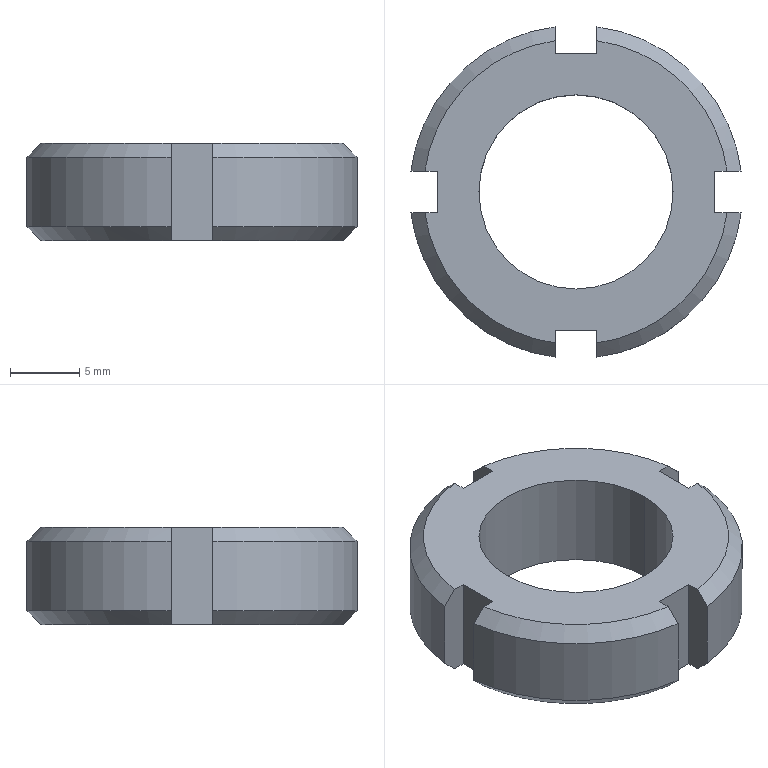Component | SolidWorks | 16RoundNutM14X1.5-1 | 1 solid | 28 faces | box 23.81 x 23.81 x 7 mm | volume 1863 mm3 | plane 14 | cone 8 | cylinder 6 | commonest cylinder face diameters 24 x4 14 x2
build123d program:
from build123d import *

# Parameters (mm, degrees)
SKETCH1_R              = 12
BOSS_EXTRUDE1_DEPTH    = 7
CHAMFER1_SIZE          = 1
M14X1_5_TAPPED_HOLE1_D = 14
SKETCH4_W              = 3
SKETCH4_H              = 4
CUT_EXTRUDE1_DEPTH     = 8
CIRPATTERN1_COUNT      = 4


with BuildPart() as part:
    # Sketch1 → Boss-Extrude1 (new body)
    with BuildSketch(Plane.XY):
        Circle(SKETCH1_R)
    extrude(amount=BOSS_EXTRUDE1_DEPTH)

    # Chamfer1
    chamfer1_edges = [part.edges().sort_by_distance(p)[0] for p in [
        (-12, 0, 0),
        (-12, 0, 7),
    ]]
    chamfer(chamfer1_edges, length=CHAMFER1_SIZE)

    # M14x1.5 Tapped Hole1 (through all)
    with Locations(Plane.XY.offset(7)):
        with Locations((0, 0)):
            Hole(M14X1_5_TAPPED_HOLE1_D / 2)

    # Sketch4 → Cut-Extrude1 (cut)
    with BuildSketch(Plane.XY):
        with Locations((0, 12)):
            Rectangle(SKETCH4_W, SKETCH4_H)
    cut_extrude1 = extrude(amount=CUT_EXTRUDE1_DEPTH, mode=Mode.SUBTRACT)

    # CirPattern1: Cut-Extrude1 ×4 about axis
    cirpattern1_axis = Axis((0, 0, 0), (0, 0, 1))
    for i in range(1, CIRPATTERN1_COUNT):
        add(cut_extrude1.rotate(cirpattern1_axis, i * 360 / CIRPATTERN1_COUNT), mode=Mode.SUBTRACT)


solid = part.part

# Placed as in the assembly
solid = solid.moved(Location((33.957, -55.224, 390), (0, 0, 0)))
STEP:
#1=COLOUR_RGB('',0.7922,0.8196,0.9333);
#2=FILL_AREA_STYLE_COLOUR('',#1);
#3=FILL_AREA_STYLE('',(#2));
#4=SURFACE_STYLE_FILL_AREA(#3);
#5=SURFACE_SIDE_STYLE('',(#4));
#6=SURFACE_STYLE_USAGE(.BOTH.,#5);
#7=PRESENTATION_STYLE_ASSIGNMENT((#6));
#8=CARTESIAN_POINT('',(1.061,-2.174,15.354));
#9=VERTEX_POINT('',#8);
#10=CARTESIAN_POINT('',(1.612,-2.174,15.354));
#11=VERTEX_POINT('',#10);
#12=CARTESIAN_POINT('',(1.337,-2.174,15.354));
#13=DIRECTION('',(0.,0.,1.));
#14=DIRECTION('',(1.,0.,0.));
#15=AXIS2_PLACEMENT_3D('',#12,#13,#14);
#16=CIRCLE('',#15,0.2756);
#17=EDGE_CURVE('',#9,#11,#16,.T.);
#18=ORIENTED_EDGE('',*,*,#17,.F.);
#19=CARTESIAN_POINT('',(1.061,-2.174,15.63));
#20=VERTEX_POINT('',#19);
#21=CARTESIAN_POINT('',(1.061,-2.174,15.63));
#22=DIRECTION('',(0.,0.,1.));
#23=VECTOR('',#22,39.37);
#24=LINE('',#21,#23);
#25=EDGE_CURVE('',#9,#20,#24,.T.);
#26=ORIENTED_EDGE('',*,*,#25,.T.);
#27=CARTESIAN_POINT('',(1.612,-2.174,15.63));
#28=VERTEX_POINT('',#27);
#29=CARTESIAN_POINT('',(1.337,-2.174,15.63));
#30=DIRECTION('',(0.,0.,1.));
#31=DIRECTION('',(1.,0.,0.));
#32=AXIS2_PLACEMENT_3D('',#29,#30,#31);
#33=CIRCLE('',#32,0.2756);
#34=EDGE_CURVE('',#20,#28,#33,.T.);
#35=ORIENTED_EDGE('',*,*,#34,.T.);
#36=CARTESIAN_POINT('',(1.612,-2.174,15.63));
#37=DIRECTION('',(0.,0.,1.));
#38=VECTOR('',#37,39.37);
#39=LINE('',#36,#38);
#40=EDGE_CURVE('',#11,#28,#39,.T.);
#41=ORIENTED_EDGE('',*,*,#40,.F.);
#42=EDGE_LOOP('',(#18,#26,#35,#41));
#43=FACE_OUTER_BOUND('',#42,.T.);
#44=CARTESIAN_POINT('',(1.337,-2.174,15.63));
#45=DIRECTION('',(0.,0.,1.));
#46=DIRECTION('',(1.,0.,0.));
#47=AXIS2_PLACEMENT_3D('',#44,#45,#46);
#48=CYLINDRICAL_SURFACE('',#47,0.2756);
#49=ADVANCED_FACE('',(#43),#48,.F.);
#50=CARTESIAN_POINT('',(1.278,-2.643,15.591));
#51=VERTEX_POINT('',#50);
#52=CARTESIAN_POINT('',(1.278,-2.643,15.394));
#53=VERTEX_POINT('',#52);
#54=CARTESIAN_POINT('',(1.278,-2.643,15.63));
#55=DIRECTION('',(0.,0.,-1.));
#56=VECTOR('',#55,39.37);
#57=LINE('',#54,#56);
#58=EDGE_CURVE('',#51,#53,#57,.T.);
#59=ORIENTED_EDGE('',*,*,#58,.F.);
#60=CARTESIAN_POINT('',(0.8682,-2.233,15.591));
#61=VERTEX_POINT('',#60);
#62=CARTESIAN_POINT('',(1.337,-2.174,15.591));
#63=DIRECTION('',(0.,0.,-1.));
#64=DIRECTION('',(1.,0.,0.));
#65=AXIS2_PLACEMENT_3D('',#62,#63,#64);
#66=CIRCLE('',#65,0.4724);
#67=EDGE_CURVE('',#51,#61,#66,.T.);
#68=ORIENTED_EDGE('',*,*,#67,.T.);
#69=CARTESIAN_POINT('',(0.8682,-2.233,15.394));
#70=VERTEX_POINT('',#69);
#71=CARTESIAN_POINT('',(0.8682,-2.233,15.63));
#72=DIRECTION('',(0.,0.,1.));
#73=VECTOR('',#72,39.37);
#74=LINE('',#71,#73);
#75=EDGE_CURVE('',#70,#61,#74,.T.);
#76=ORIENTED_EDGE('',*,*,#75,.F.);
#77=CARTESIAN_POINT('',(1.337,-2.174,15.394));
#78=DIRECTION('',(0.,0.,1.));
#79=DIRECTION('',(1.,0.,0.));
#80=AXIS2_PLACEMENT_3D('',#77,#78,#79);
#81=CIRCLE('',#80,0.4724);
#82=EDGE_CURVE('',#70,#53,#81,.T.);
#83=ORIENTED_EDGE('',*,*,#82,.T.);
#84=EDGE_LOOP('',(#59,#68,#76,#83));
#85=FACE_OUTER_BOUND('',#84,.T.);
#86=CARTESIAN_POINT('',(1.337,-2.174,15.63));
#87=DIRECTION('',(0.,0.,-1.));
#88=DIRECTION('',(-1.,0.,0.));
#89=AXIS2_PLACEMENT_3D('',#86,#87,#88);
#90=CYLINDRICAL_SURFACE('',#89,0.4724);
#91=ADVANCED_FACE('',(#85),#90,.T.);
#92=CARTESIAN_POINT('',(1.396,-2.643,15.394));
#93=VERTEX_POINT('',#92);
#94=CARTESIAN_POINT('',(1.396,-2.643,15.591));
#95=VERTEX_POINT('',#94);
#96=CARTESIAN_POINT('',(1.396,-2.643,15.63));
#97=DIRECTION('',(0.,0.,1.));
#98=VECTOR('',#97,39.37);
#99=LINE('',#96,#98);
#100=EDGE_CURVE('',#93,#95,#99,.T.);
#101=ORIENTED_EDGE('',*,*,#100,.F.);
#102=CARTESIAN_POINT('',(1.806,-2.233,15.394));
#103=VERTEX_POINT('',#102);
#104=CARTESIAN_POINT('',(1.337,-2.174,15.394));
#105=DIRECTION('',(0.,0.,1.));
#106=DIRECTION('',(1.,0.,0.));
#107=AXIS2_PLACEMENT_3D('',#104,#105,#106);
#108=CIRCLE('',#107,0.4724);
#109=EDGE_CURVE('',#93,#103,#108,.T.);
#110=ORIENTED_EDGE('',*,*,#109,.T.);
#111=CARTESIAN_POINT('',(1.806,-2.233,15.591));
#112=VERTEX_POINT('',#111);
#113=CARTESIAN_POINT('',(1.806,-2.233,15.63));
#114=DIRECTION('',(0.,0.,-1.));
#115=VECTOR('',#114,39.37);
#116=LINE('',#113,#115);
#117=EDGE_CURVE('',#112,#103,#116,.T.);
#118=ORIENTED_EDGE('',*,*,#117,.F.);
#119=CARTESIAN_POINT('',(1.337,-2.174,15.591));
#120=DIRECTION('',(0.,0.,-1.));
#121=DIRECTION('',(1.,0.,0.));
#122=AXIS2_PLACEMENT_3D('',#119,#120,#121);
#123=CIRCLE('',#122,0.4724);
#124=EDGE_CURVE('',#112,#95,#123,.T.);
#125=ORIENTED_EDGE('',*,*,#124,.T.);
#126=EDGE_LOOP('',(#101,#110,#118,#125));
#127=FACE_OUTER_BOUND('',#126,.T.);
#128=CARTESIAN_POINT('',(1.337,-2.174,15.63));
#129=DIRECTION('',(0.,0.,-1.));
#130=DIRECTION('',(-1.,0.,0.));
#131=AXIS2_PLACEMENT_3D('',#128,#129,#130);
#132=CYLINDRICAL_SURFACE('',#131,0.4724);
#133=ADVANCED_FACE('',(#127),#132,.T.);
#134=CARTESIAN_POINT('',(0.8682,-2.115,15.591));
#135=VERTEX_POINT('',#134);
#136=CARTESIAN_POINT('',(0.8682,-2.115,15.394));
#137=VERTEX_POINT('',#136);
#138=CARTESIAN_POINT('',(0.8682,-2.115,15.63));
#139=DIRECTION('',(0.,0.,-1.));
#140=VECTOR('',#139,39.37);
#141=LINE('',#138,#140);
#142=EDGE_CURVE('',#135,#137,#141,.T.);
#143=ORIENTED_EDGE('',*,*,#142,.F.);
#144=CARTESIAN_POINT('',(1.278,-1.705,15.591));
#145=VERTEX_POINT('',#144);
#146=CARTESIAN_POINT('',(1.337,-2.174,15.591));
#147=DIRECTION('',(0.,0.,-1.));
#148=DIRECTION('',(1.,0.,0.));
#149=AXIS2_PLACEMENT_3D('',#146,#147,#148);
#150=CIRCLE('',#149,0.4724);
#151=EDGE_CURVE('',#135,#145,#150,.T.);
#152=ORIENTED_EDGE('',*,*,#151,.T.);
#153=CARTESIAN_POINT('',(1.278,-1.705,15.394));
#154=VERTEX_POINT('',#153);
#155=CARTESIAN_POINT('',(1.278,-1.705,15.63));
#156=DIRECTION('',(0.,0.,1.));
#157=VECTOR('',#156,39.37);
#158=LINE('',#155,#157);
#159=EDGE_CURVE('',#154,#145,#158,.T.);
#160=ORIENTED_EDGE('',*,*,#159,.F.);
#161=CARTESIAN_POINT('',(1.337,-2.174,15.394));
#162=DIRECTION('',(0.,0.,1.));
#163=DIRECTION('',(1.,0.,0.));
#164=AXIS2_PLACEMENT_3D('',#161,#162,#163);
#165=CIRCLE('',#164,0.4724);
#166=EDGE_CURVE('',#154,#137,#165,.T.);
#167=ORIENTED_EDGE('',*,*,#166,.T.);
#168=EDGE_LOOP('',(#143,#152,#160,#167));
#169=FACE_OUTER_BOUND('',#168,.T.);
#170=CARTESIAN_POINT('',(1.337,-2.174,15.63));
#171=DIRECTION('',(0.,0.,-1.));
#172=DIRECTION('',(-1.,0.,0.));
#173=AXIS2_PLACEMENT_3D('',#170,#171,#172);
#174=CYLINDRICAL_SURFACE('',#173,0.4724);
#175=ADVANCED_FACE('',(#169),#174,.T.);
#176=CARTESIAN_POINT('',(1.337,-2.174,15.63));
#177=DIRECTION('',(0.,0.,1.));
#178=DIRECTION('',(1.,0.,0.));
#179=AXIS2_PLACEMENT_3D('',#176,#177,#178);
#180=CIRCLE('',#179,0.2756);
#181=EDGE_CURVE('',#28,#20,#180,.T.);
#182=ORIENTED_EDGE('',*,*,#181,.F.);
#183=ORIENTED_EDGE('',*,*,#34,.F.);
#184=EDGE_LOOP('',(#182,#183));
#185=FACE_BOUND('',#184,.T.);
#186=CARTESIAN_POINT('',(0.9079,-2.233,15.63));
#187=VERTEX_POINT('',#186);
#188=CARTESIAN_POINT('',(1.278,-2.603,15.63));
#189=VERTEX_POINT('',#188);
#190=CARTESIAN_POINT('',(1.337,-2.174,15.63));
#191=DIRECTION('',(0.,0.,1.));
#192=DIRECTION('',(1.,0.,0.));
#193=AXIS2_PLACEMENT_3D('',#190,#191,#192);
#194=CIRCLE('',#193,0.4331);
#195=EDGE_CURVE('',#187,#189,#194,.T.);
#196=ORIENTED_EDGE('',*,*,#195,.T.);
#197=CARTESIAN_POINT('',(1.278,-2.568,15.63));
#198=VERTEX_POINT('',#197);
#199=CARTESIAN_POINT('',(1.278,-2.174,15.63));
#200=DIRECTION('',(0.,1.,0.));
#201=VECTOR('',#200,39.37);
#202=LINE('',#199,#201);
#203=EDGE_CURVE('',#189,#198,#202,.T.);
#204=ORIENTED_EDGE('',*,*,#203,.T.);
#205=CARTESIAN_POINT('',(1.396,-2.568,15.63));
#206=VERTEX_POINT('',#205);
#207=CARTESIAN_POINT('',(1.337,-2.568,15.63));
#208=DIRECTION('',(1.,0.,0.));
#209=VECTOR('',#208,39.37);
#210=LINE('',#207,#209);
#211=EDGE_CURVE('',#198,#206,#210,.T.);
#212=ORIENTED_EDGE('',*,*,#211,.T.);
#213=CARTESIAN_POINT('',(1.396,-2.603,15.63));
#214=VERTEX_POINT('',#213);
#215=CARTESIAN_POINT('',(1.396,-2.174,15.63));
#216=DIRECTION('',(-0.,-1.,0.));
#217=VECTOR('',#216,39.37);
#218=LINE('',#215,#217);
#219=EDGE_CURVE('',#206,#214,#218,.T.);
#220=ORIENTED_EDGE('',*,*,#219,.T.);
#221=CARTESIAN_POINT('',(1.766,-2.233,15.63));
#222=VERTEX_POINT('',#221);
#223=CARTESIAN_POINT('',(1.337,-2.174,15.63));
#224=DIRECTION('',(0.,0.,1.));
#225=DIRECTION('',(1.,0.,0.));
#226=AXIS2_PLACEMENT_3D('',#223,#224,#225);
#227=CIRCLE('',#226,0.4331);
#228=EDGE_CURVE('',#214,#222,#227,.T.);
#229=ORIENTED_EDGE('',*,*,#228,.T.);
#230=CARTESIAN_POINT('',(1.731,-2.233,15.63));
#231=VERTEX_POINT('',#230);
#232=CARTESIAN_POINT('',(1.337,-2.233,15.63));
#233=DIRECTION('',(-1.,0.,0.));
#234=VECTOR('',#233,39.37);
#235=LINE('',#232,#234);
#236=EDGE_CURVE('',#222,#231,#235,.T.);
#237=ORIENTED_EDGE('',*,*,#236,.T.);
#238=CARTESIAN_POINT('',(1.731,-2.115,15.63));
#239=VERTEX_POINT('',#238);
#240=CARTESIAN_POINT('',(1.731,-2.174,15.63));
#241=DIRECTION('',(0.,1.,0.));
#242=VECTOR('',#241,39.37);
#243=LINE('',#240,#242);
#244=EDGE_CURVE('',#231,#239,#243,.T.);
#245=ORIENTED_EDGE('',*,*,#244,.T.);
#246=CARTESIAN_POINT('',(1.766,-2.115,15.63));
#247=VERTEX_POINT('',#246);
#248=CARTESIAN_POINT('',(1.337,-2.115,15.63));
#249=DIRECTION('',(1.,-0.,0.));
#250=VECTOR('',#249,39.37);
#251=LINE('',#248,#250);
#252=EDGE_CURVE('',#239,#247,#251,.T.);
#253=ORIENTED_EDGE('',*,*,#252,.T.);
#254=CARTESIAN_POINT('',(1.396,-1.745,15.63));
#255=VERTEX_POINT('',#254);
#256=CARTESIAN_POINT('',(1.337,-2.174,15.63));
#257=DIRECTION('',(0.,0.,1.));
#258=DIRECTION('',(1.,0.,0.));
#259=AXIS2_PLACEMENT_3D('',#256,#257,#258);
#260=CIRCLE('',#259,0.4331);
#261=EDGE_CURVE('',#247,#255,#260,.T.);
#262=ORIENTED_EDGE('',*,*,#261,.T.);
#263=CARTESIAN_POINT('',(1.396,-1.78,15.63));
#264=VERTEX_POINT('',#263);
#265=CARTESIAN_POINT('',(1.396,-2.174,15.63));
#266=DIRECTION('',(-0.,-1.,0.));
#267=VECTOR('',#266,39.37);
#268=LINE('',#265,#267);
#269=EDGE_CURVE('',#255,#264,#268,.T.);
#270=ORIENTED_EDGE('',*,*,#269,.T.);
#271=CARTESIAN_POINT('',(1.278,-1.78,15.63));
#272=VERTEX_POINT('',#271);
#273=CARTESIAN_POINT('',(1.337,-1.78,15.63));
#274=DIRECTION('',(-1.,0.,0.));
#275=VECTOR('',#274,39.37);
#276=LINE('',#273,#275);
#277=EDGE_CURVE('',#264,#272,#276,.T.);
#278=ORIENTED_EDGE('',*,*,#277,.T.);
#279=CARTESIAN_POINT('',(1.278,-1.745,15.63));
#280=VERTEX_POINT('',#279);
#281=CARTESIAN_POINT('',(1.278,-2.174,15.63));
#282=DIRECTION('',(0.,1.,0.));
#283=VECTOR('',#282,39.37);
#284=LINE('',#281,#283);
#285=EDGE_CURVE('',#272,#280,#284,.T.);
#286=ORIENTED_EDGE('',*,*,#285,.T.);
#287=CARTESIAN_POINT('',(0.9079,-2.115,15.63));
#288=VERTEX_POINT('',#287);
#289=CARTESIAN_POINT('',(1.337,-2.174,15.63));
#290=DIRECTION('',(0.,0.,1.));
#291=DIRECTION('',(1.,0.,0.));
#292=AXIS2_PLACEMENT_3D('',#289,#290,#291);
#293=CIRCLE('',#292,0.4331);
#294=EDGE_CURVE('',#280,#288,#293,.T.);
#295=ORIENTED_EDGE('',*,*,#294,.T.);
#296=CARTESIAN_POINT('',(0.9432,-2.115,15.63));
#297=VERTEX_POINT('',#296);
#298=CARTESIAN_POINT('',(1.337,-2.115,15.63));
#299=DIRECTION('',(1.,-0.,0.));
#300=VECTOR('',#299,39.37);
#301=LINE('',#298,#300);
#302=EDGE_CURVE('',#288,#297,#301,.T.);
#303=ORIENTED_EDGE('',*,*,#302,.T.);
#304=CARTESIAN_POINT('',(0.9432,-2.233,15.63));
#305=VERTEX_POINT('',#304);
#306=CARTESIAN_POINT('',(0.9432,-2.174,15.63));
#307=DIRECTION('',(-0.,-1.,0.));
#308=VECTOR('',#307,39.37);
#309=LINE('',#306,#308);
#310=EDGE_CURVE('',#297,#305,#309,.T.);
#311=ORIENTED_EDGE('',*,*,#310,.T.);
#312=CARTESIAN_POINT('',(1.337,-2.233,15.63));
#313=DIRECTION('',(-1.,0.,0.));
#314=VECTOR('',#313,39.37);
#315=LINE('',#312,#314);
#316=EDGE_CURVE('',#305,#187,#315,.T.);
#317=ORIENTED_EDGE('',*,*,#316,.T.);
#318=EDGE_LOOP('',(#196,#204,#212,#220,#229,#237,#245,#253,#262,#270,#278,#286,#295,#303,#311,#317));
#319=FACE_OUTER_BOUND('',#318,.T.);
#320=CARTESIAN_POINT('',(1.337,-2.174,15.63));
#321=DIRECTION('',(0.,0.,1.));
#322=DIRECTION('',(1.,0.,0.));
#323=AXIS2_PLACEMENT_3D('',#320,#321,#322);
#324=PLANE('',#323);
#325=ADVANCED_FACE('',(#185,#319),#324,.T.);
#326=CARTESIAN_POINT('',(1.337,-2.174,15.354));
#327=DIRECTION('',(0.,0.,1.));
#328=DIRECTION('',(1.,0.,0.));
#329=AXIS2_PLACEMENT_3D('',#326,#327,#328);
#330=CIRCLE('',#329,0.2756);
#331=EDGE_CURVE('',#11,#9,#330,.T.);
#332=ORIENTED_EDGE('',*,*,#331,.T.);
#333=ORIENTED_EDGE('',*,*,#17,.T.);
#334=EDGE_LOOP('',(#332,#333));
#335=FACE_BOUND('',#334,.T.);
#336=CARTESIAN_POINT('',(1.278,-2.568,15.354));
#337=VERTEX_POINT('',#336);
#338=CARTESIAN_POINT('',(1.278,-2.603,15.354));
#339=VERTEX_POINT('',#338);
#340=CARTESIAN_POINT('',(1.278,-2.568,15.354));
#341=DIRECTION('',(-0.,-1.,0.));
#342=VECTOR('',#341,39.37);
#343=LINE('',#340,#342);
#344=EDGE_CURVE('',#337,#339,#343,.T.);
#345=ORIENTED_EDGE('',*,*,#344,.T.);
#346=CARTESIAN_POINT('',(0.9079,-2.233,15.354));
#347=VERTEX_POINT('',#346);
#348=CARTESIAN_POINT('',(1.337,-2.174,15.354));
#349=DIRECTION('',(0.,0.,-1.));
#350=DIRECTION('',(1.,0.,0.));
#351=AXIS2_PLACEMENT_3D('',#348,#349,#350);
#352=CIRCLE('',#351,0.4331);
#353=EDGE_CURVE('',#339,#347,#352,.T.);
#354=ORIENTED_EDGE('',*,*,#353,.T.);
#355=CARTESIAN_POINT('',(0.9432,-2.233,15.354));
#356=VERTEX_POINT('',#355);
#357=CARTESIAN_POINT('',(0.9432,-2.233,15.354));
#358=DIRECTION('',(1.,-0.,0.));
#359=VECTOR('',#358,39.37);
#360=LINE('',#357,#359);
#361=EDGE_CURVE('',#347,#356,#360,.T.);
#362=ORIENTED_EDGE('',*,*,#361,.T.);
#363=CARTESIAN_POINT('',(0.9432,-2.115,15.354));
#364=VERTEX_POINT('',#363);
#365=CARTESIAN_POINT('',(0.9432,-2.233,15.354));
#366=DIRECTION('',(0.,1.,0.));
#367=VECTOR('',#366,39.37);
#368=LINE('',#365,#367);
#369=EDGE_CURVE('',#356,#364,#368,.T.);
#370=ORIENTED_EDGE('',*,*,#369,.T.);
#371=CARTESIAN_POINT('',(0.9079,-2.115,15.354));
#372=VERTEX_POINT('',#371);
#373=CARTESIAN_POINT('',(0.9432,-2.115,15.354));
#374=DIRECTION('',(-1.,0.,0.));
#375=VECTOR('',#374,39.37);
#376=LINE('',#373,#375);
#377=EDGE_CURVE('',#364,#372,#376,.T.);
#378=ORIENTED_EDGE('',*,*,#377,.T.);
#379=CARTESIAN_POINT('',(1.278,-1.745,15.354));
#380=VERTEX_POINT('',#379);
#381=CARTESIAN_POINT('',(1.337,-2.174,15.354));
#382=DIRECTION('',(0.,0.,-1.));
#383=DIRECTION('',(1.,0.,0.));
#384=AXIS2_PLACEMENT_3D('',#381,#382,#383);
#385=CIRCLE('',#384,0.4331);
#386=EDGE_CURVE('',#372,#380,#385,.T.);
#387=ORIENTED_EDGE('',*,*,#386,.T.);
#388=CARTESIAN_POINT('',(1.278,-1.78,15.354));
#389=VERTEX_POINT('',#388);
#390=CARTESIAN_POINT('',(1.278,-1.78,15.354));
#391=DIRECTION('',(-0.,-1.,0.));
#392=VECTOR('',#391,39.37);
#393=LINE('',#390,#392);
#394=EDGE_CURVE('',#380,#389,#393,.T.);
#395=ORIENTED_EDGE('',*,*,#394,.T.);
#396=CARTESIAN_POINT('',(1.396,-1.78,15.354));
#397=VERTEX_POINT('',#396);
#398=CARTESIAN_POINT('',(1.278,-1.78,15.354));
#399=DIRECTION('',(1.,0.,0.));
#400=VECTOR('',#399,39.37);
#401=LINE('',#398,#400);
#402=EDGE_CURVE('',#389,#397,#401,.T.);
#403=ORIENTED_EDGE('',*,*,#402,.T.);
#404=CARTESIAN_POINT('',(1.396,-1.745,15.354));
#405=VERTEX_POINT('',#404);
#406=CARTESIAN_POINT('',(1.396,-1.78,15.354));
#407=DIRECTION('',(0.,1.,0.));
#408=VECTOR('',#407,39.37);
#409=LINE('',#406,#408);
#410=EDGE_CURVE('',#397,#405,#409,.T.);
#411=ORIENTED_EDGE('',*,*,#410,.T.);
#412=CARTESIAN_POINT('',(1.766,-2.115,15.354));
#413=VERTEX_POINT('',#412);
#414=CARTESIAN_POINT('',(1.337,-2.174,15.354));
#415=DIRECTION('',(0.,0.,-1.));
#416=DIRECTION('',(1.,-0.,0.));
#417=AXIS2_PLACEMENT_3D('',#414,#415,#416);
#418=CIRCLE('',#417,0.4331);
#419=EDGE_CURVE('',#405,#413,#418,.T.);
#420=ORIENTED_EDGE('',*,*,#419,.T.);
#421=CARTESIAN_POINT('',(1.731,-2.115,15.354));
#422=VERTEX_POINT('',#421);
#423=CARTESIAN_POINT('',(1.731,-2.115,15.354));
#424=DIRECTION('',(-1.,0.,0.));
#425=VECTOR('',#424,39.37);
#426=LINE('',#423,#425);
#427=EDGE_CURVE('',#413,#422,#426,.T.);
#428=ORIENTED_EDGE('',*,*,#427,.T.);
#429=CARTESIAN_POINT('',(1.731,-2.233,15.354));
#430=VERTEX_POINT('',#429);
#431=CARTESIAN_POINT('',(1.731,-2.115,15.354));
#432=DIRECTION('',(-0.,-1.,0.));
#433=VECTOR('',#432,39.37);
#434=LINE('',#431,#433);
#435=EDGE_CURVE('',#422,#430,#434,.T.);
#436=ORIENTED_EDGE('',*,*,#435,.T.);
#437=CARTESIAN_POINT('',(1.766,-2.233,15.354));
#438=VERTEX_POINT('',#437);
#439=CARTESIAN_POINT('',(1.731,-2.233,15.354));
#440=DIRECTION('',(1.,-0.,0.));
#441=VECTOR('',#440,39.37);
#442=LINE('',#439,#441);
#443=EDGE_CURVE('',#430,#438,#442,.T.);
#444=ORIENTED_EDGE('',*,*,#443,.T.);
#445=CARTESIAN_POINT('',(1.396,-2.603,15.354));
#446=VERTEX_POINT('',#445);
#447=CARTESIAN_POINT('',(1.337,-2.174,15.354));
#448=DIRECTION('',(0.,0.,-1.));
#449=DIRECTION('',(1.,0.,0.));
#450=AXIS2_PLACEMENT_3D('',#447,#448,#449);
#451=CIRCLE('',#450,0.4331);
#452=EDGE_CURVE('',#438,#446,#451,.T.);
#453=ORIENTED_EDGE('',*,*,#452,.T.);
#454=CARTESIAN_POINT('',(1.396,-2.568,15.354));
#455=VERTEX_POINT('',#454);
#456=CARTESIAN_POINT('',(1.396,-2.568,15.354));
#457=DIRECTION('',(0.,1.,0.));
#458=VECTOR('',#457,39.37);
#459=LINE('',#456,#458);
#460=EDGE_CURVE('',#446,#455,#459,.T.);
#461=ORIENTED_EDGE('',*,*,#460,.T.);
#462=CARTESIAN_POINT('',(1.396,-2.568,15.354));
#463=DIRECTION('',(-1.,0.,0.));
#464=VECTOR('',#463,39.37);
#465=LINE('',#462,#464);
#466=EDGE_CURVE('',#455,#337,#465,.T.);
#467=ORIENTED_EDGE('',*,*,#466,.T.);
#468=EDGE_LOOP('',(#345,#354,#362,#370,#378,#387,#395,#403,#411,#420,#428,#436,#444,#453,#461,#467));
#469=FACE_OUTER_BOUND('',#468,.T.);
#470=CARTESIAN_POINT('',(1.337,-2.174,15.354));
#471=DIRECTION('',(0.,0.,1.));
#472=DIRECTION('',(1.,0.,0.));
#473=AXIS2_PLACEMENT_3D('',#470,#471,#472);
#474=PLANE('',#473);
#475=ADVANCED_FACE('',(#335,#469),#474,.F.);
#476=ORIENTED_EDGE('',*,*,#353,.F.);
#477=CARTESIAN_POINT('',(1.278,-2.603,15.354));
#478=CARTESIAN_POINT('',(1.278,-2.616,15.367));
#479=CARTESIAN_POINT('',(1.278,-2.63,15.381));
#480=CARTESIAN_POINT('',(1.278,-2.643,15.394));
#481=B_SPLINE_CURVE_WITH_KNOTS('',3,(#477,#478,#479,#480),.UNSPECIFIED.,.F.,.F.,(4,4),(0.004369,0.00579),.UNSPECIFIED.);
#482=EDGE_CURVE('',#339,#53,#481,.T.);
#483=ORIENTED_EDGE('',*,*,#482,.T.);
#484=ORIENTED_EDGE('',*,*,#82,.F.);
#485=CARTESIAN_POINT('',(0.8682,-2.233,15.394));
#486=CARTESIAN_POINT('',(0.8814,-2.233,15.381));
#487=CARTESIAN_POINT('',(0.8946,-2.233,15.367));
#488=CARTESIAN_POINT('',(0.9079,-2.233,15.354));
#489=B_SPLINE_CURVE_WITH_KNOTS('',3,(#485,#486,#487,#488),.UNSPECIFIED.,.F.,.F.,(4,4),(0.003092,0.004512),.UNSPECIFIED.);
#490=EDGE_CURVE('',#70,#347,#489,.T.);
#491=ORIENTED_EDGE('',*,*,#490,.T.);
#492=EDGE_LOOP('',(#476,#483,#484,#491));
#493=FACE_OUTER_BOUND('',#492,.T.);
#494=CARTESIAN_POINT('',(1.337,-2.174,15.394));
#495=DIRECTION('',(0.,0.,1.));
#496=DIRECTION('',(1.,0.,0.));
#497=AXIS2_PLACEMENT_3D('',#494,#495,#496);
#498=CONICAL_SURFACE('',#497,0.4724,0.7854);
#499=ADVANCED_FACE('',(#493),#498,.T.);
#500=ORIENTED_EDGE('',*,*,#109,.F.);
#501=CARTESIAN_POINT('',(1.396,-2.643,15.394));
#502=CARTESIAN_POINT('',(1.396,-2.63,15.381));
#503=CARTESIAN_POINT('',(1.396,-2.616,15.367));
#504=CARTESIAN_POINT('',(1.396,-2.603,15.354));
#505=B_SPLINE_CURVE_WITH_KNOTS('',3,(#501,#502,#503,#504),.UNSPECIFIED.,.F.,.F.,(4,4),(0.003092,0.004512),.UNSPECIFIED.);
#506=EDGE_CURVE('',#93,#446,#505,.T.);
#507=ORIENTED_EDGE('',*,*,#506,.T.);
#508=ORIENTED_EDGE('',*,*,#452,.F.);
#509=CARTESIAN_POINT('',(1.766,-2.233,15.354));
#510=CARTESIAN_POINT('',(1.779,-2.233,15.367));
#511=CARTESIAN_POINT('',(1.792,-2.233,15.381));
#512=CARTESIAN_POINT('',(1.806,-2.233,15.394));
#513=B_SPLINE_CURVE_WITH_KNOTS('',3,(#509,#510,#511,#512),.UNSPECIFIED.,.F.,.F.,(4,4),(0.004369,0.00579),.UNSPECIFIED.);
#514=EDGE_CURVE('',#438,#103,#513,.T.);
#515=ORIENTED_EDGE('',*,*,#514,.T.);
#516=EDGE_LOOP('',(#500,#507,#508,#515));
#517=FACE_OUTER_BOUND('',#516,.T.);
#518=CARTESIAN_POINT('',(1.337,-2.174,15.394));
#519=DIRECTION('',(0.,0.,1.));
#520=DIRECTION('',(1.,0.,0.));
#521=AXIS2_PLACEMENT_3D('',#518,#519,#520);
#522=CONICAL_SURFACE('',#521,0.4724,0.7854);
#523=ADVANCED_FACE('',(#517),#522,.T.);
#524=ORIENTED_EDGE('',*,*,#386,.F.);
#525=CARTESIAN_POINT('',(0.9079,-2.115,15.354));
#526=CARTESIAN_POINT('',(0.8946,-2.115,15.367));
#527=CARTESIAN_POINT('',(0.8814,-2.115,15.381));
#528=CARTESIAN_POINT('',(0.8682,-2.115,15.394));
#529=B_SPLINE_CURVE_WITH_KNOTS('',3,(#525,#526,#527,#528),.UNSPECIFIED.,.F.,.F.,(4,4),(0.004369,0.00579),.UNSPECIFIED.);
#530=EDGE_CURVE('',#372,#137,#529,.T.);
#531=ORIENTED_EDGE('',*,*,#530,.T.);
#532=ORIENTED_EDGE('',*,*,#166,.F.);
#533=CARTESIAN_POINT('',(1.278,-1.705,15.394));
#534=CARTESIAN_POINT('',(1.278,-1.719,15.381));
#535=CARTESIAN_POINT('',(1.278,-1.732,15.367));
#536=CARTESIAN_POINT('',(1.278,-1.745,15.354));
#537=B_SPLINE_CURVE_WITH_KNOTS('',3,(#533,#534,#535,#536),.UNSPECIFIED.,.F.,.F.,(4,4),(0.003092,0.004512),.UNSPECIFIED.);
#538=EDGE_CURVE('',#154,#380,#537,.T.);
#539=ORIENTED_EDGE('',*,*,#538,.T.);
#540=EDGE_LOOP('',(#524,#531,#532,#539));
#541=FACE_OUTER_BOUND('',#540,.T.);
#542=CARTESIAN_POINT('',(1.337,-2.174,15.394));
#543=DIRECTION('',(0.,0.,1.));
#544=DIRECTION('',(1.,0.,0.));
#545=AXIS2_PLACEMENT_3D('',#542,#543,#544);
#546=CONICAL_SURFACE('',#545,0.4724,0.7854);
#547=ADVANCED_FACE('',(#541),#546,.T.);
#548=ORIENTED_EDGE('',*,*,#67,.F.);
#549=CARTESIAN_POINT('',(1.278,-2.643,15.591));
#550=CARTESIAN_POINT('',(1.278,-2.63,15.604));
#551=CARTESIAN_POINT('',(1.278,-2.616,15.617));
#552=CARTESIAN_POINT('',(1.278,-2.603,15.63));
#553=B_SPLINE_CURVE_WITH_KNOTS('',3,(#549,#550,#551,#552),.UNSPECIFIED.,.F.,.F.,(4,4),(0.003092,0.004512),.UNSPECIFIED.);
#554=EDGE_CURVE('',#51,#189,#553,.T.);
#555=ORIENTED_EDGE('',*,*,#554,.T.);
#556=ORIENTED_EDGE('',*,*,#195,.F.);
#557=CARTESIAN_POINT('',(0.9079,-2.233,15.63));
#558=CARTESIAN_POINT('',(0.8946,-2.233,15.617));
#559=CARTESIAN_POINT('',(0.8814,-2.233,15.604));
#560=CARTESIAN_POINT('',(0.8682,-2.233,15.591));
#561=B_SPLINE_CURVE_WITH_KNOTS('',3,(#557,#558,#559,#560),.UNSPECIFIED.,.F.,.F.,(4,4),(0.004369,0.00579),.UNSPECIFIED.);
#562=EDGE_CURVE('',#187,#61,#561,.T.);
#563=ORIENTED_EDGE('',*,*,#562,.T.);
#564=EDGE_LOOP('',(#548,#555,#556,#563));
#565=FACE_OUTER_BOUND('',#564,.T.);
#566=CARTESIAN_POINT('',(1.337,-2.174,15.63));
#567=DIRECTION('',(0.,0.,-1.));
#568=DIRECTION('',(-1.,0.,0.));
#569=AXIS2_PLACEMENT_3D('',#566,#567,#568);
#570=CONICAL_SURFACE('',#569,0.4331,0.7854);
#571=ADVANCED_FACE('',(#565),#570,.T.);
#572=ORIENTED_EDGE('',*,*,#228,.F.);
#573=CARTESIAN_POINT('',(1.396,-2.603,15.63));
#574=CARTESIAN_POINT('',(1.396,-2.616,15.617));
#575=CARTESIAN_POINT('',(1.396,-2.63,15.604));
#576=CARTESIAN_POINT('',(1.396,-2.643,15.591));
#577=B_SPLINE_CURVE_WITH_KNOTS('',3,(#573,#574,#575,#576),.UNSPECIFIED.,.F.,.F.,(4,4),(0.004369,0.00579),.UNSPECIFIED.);
#578=EDGE_CURVE('',#214,#95,#577,.T.);
#579=ORIENTED_EDGE('',*,*,#578,.T.);
#580=ORIENTED_EDGE('',*,*,#124,.F.);
#581=CARTESIAN_POINT('',(1.806,-2.233,15.591));
#582=CARTESIAN_POINT('',(1.792,-2.233,15.604));
#583=CARTESIAN_POINT('',(1.779,-2.233,15.617));
#584=CARTESIAN_POINT('',(1.766,-2.233,15.63));
#585=B_SPLINE_CURVE_WITH_KNOTS('',3,(#581,#582,#583,#584),.UNSPECIFIED.,.F.,.F.,(4,4),(0.003092,0.004512),.UNSPECIFIED.);
#586=EDGE_CURVE('',#112,#222,#585,.T.);
#587=ORIENTED_EDGE('',*,*,#586,.T.);
#588=EDGE_LOOP('',(#572,#579,#580,#587));
#589=FACE_OUTER_BOUND('',#588,.T.);
#590=CARTESIAN_POINT('',(1.337,-2.174,15.63));
#591=DIRECTION('',(0.,0.,-1.));
#592=DIRECTION('',(-1.,0.,0.));
#593=AXIS2_PLACEMENT_3D('',#590,#591,#592);
#594=CONICAL_SURFACE('',#593,0.4331,0.7854);
#595=ADVANCED_FACE('',(#589),#594,.T.);
#596=ORIENTED_EDGE('',*,*,#151,.F.);
#597=CARTESIAN_POINT('',(0.8682,-2.115,15.591));
#598=CARTESIAN_POINT('',(0.8814,-2.115,15.604));
#599=CARTESIAN_POINT('',(0.8946,-2.115,15.617));
#600=CARTESIAN_POINT('',(0.9079,-2.115,15.63));
#601=B_SPLINE_CURVE_WITH_KNOTS('',3,(#597,#598,#599,#600),.UNSPECIFIED.,.F.,.F.,(4,4),(0.003092,0.004512),.UNSPECIFIED.);
#602=EDGE_CURVE('',#135,#288,#601,.T.);
#603=ORIENTED_EDGE('',*,*,#602,.T.);
#604=ORIENTED_EDGE('',*,*,#294,.F.);
#605=CARTESIAN_POINT('',(1.278,-1.745,15.63));
#606=CARTESIAN_POINT('',(1.278,-1.732,15.617));
#607=CARTESIAN_POINT('',(1.278,-1.719,15.604));
#608=CARTESIAN_POINT('',(1.278,-1.705,15.591));
#609=B_SPLINE_CURVE_WITH_KNOTS('',3,(#605,#606,#607,#608),.UNSPECIFIED.,.F.,.F.,(4,4),(0.004369,0.00579),.UNSPECIFIED.);
#610=EDGE_CURVE('',#280,#145,#609,.T.);
#611=ORIENTED_EDGE('',*,*,#610,.T.);
#612=EDGE_LOOP('',(#596,#603,#604,#611));
#613=FACE_OUTER_BOUND('',#612,.T.);
#614=CARTESIAN_POINT('',(1.337,-2.174,15.63));
#615=DIRECTION('',(0.,0.,-1.));
#616=DIRECTION('',(-1.,0.,0.));
#617=AXIS2_PLACEMENT_3D('',#614,#615,#616);
#618=CONICAL_SURFACE('',#617,0.4331,0.7854);
#619=ADVANCED_FACE('',(#613),#618,.T.);
#620=CARTESIAN_POINT('',(1.806,-2.115,15.394));
#621=VERTEX_POINT('',#620);
#622=CARTESIAN_POINT('',(1.806,-2.115,15.591));
#623=VERTEX_POINT('',#622);
#624=CARTESIAN_POINT('',(1.806,-2.115,15.63));
#625=DIRECTION('',(0.,0.,1.));
#626=VECTOR('',#625,39.37);
#627=LINE('',#624,#626);
#628=EDGE_CURVE('',#621,#623,#627,.T.);
#629=ORIENTED_EDGE('',*,*,#628,.F.);
#630=CARTESIAN_POINT('',(1.396,-1.705,15.394));
#631=VERTEX_POINT('',#630);
#632=CARTESIAN_POINT('',(1.337,-2.174,15.394));
#633=DIRECTION('',(0.,0.,1.));
#634=DIRECTION('',(1.,0.,0.));
#635=AXIS2_PLACEMENT_3D('',#632,#633,#634);
#636=CIRCLE('',#635,0.4724);
#637=EDGE_CURVE('',#621,#631,#636,.T.);
#638=ORIENTED_EDGE('',*,*,#637,.T.);
#639=CARTESIAN_POINT('',(1.396,-1.705,15.591));
#640=VERTEX_POINT('',#639);
#641=CARTESIAN_POINT('',(1.396,-1.705,15.63));
#642=DIRECTION('',(0.,0.,-1.));
#643=VECTOR('',#642,39.37);
#644=LINE('',#641,#643);
#645=EDGE_CURVE('',#640,#631,#644,.T.);
#646=ORIENTED_EDGE('',*,*,#645,.F.);
#647=CARTESIAN_POINT('',(1.337,-2.174,15.591));
#648=DIRECTION('',(0.,0.,-1.));
#649=DIRECTION('',(1.,0.,0.));
#650=AXIS2_PLACEMENT_3D('',#647,#648,#649);
#651=CIRCLE('',#650,0.4724);
#652=EDGE_CURVE('',#640,#623,#651,.T.);
#653=ORIENTED_EDGE('',*,*,#652,.T.);
#654=EDGE_LOOP('',(#629,#638,#646,#653));
#655=FACE_OUTER_BOUND('',#654,.T.);
#656=CARTESIAN_POINT('',(1.337,-2.174,15.63));
#657=DIRECTION('',(0.,0.,-1.));
#658=DIRECTION('',(-1.,0.,0.));
#659=AXIS2_PLACEMENT_3D('',#656,#657,#658);
#660=CYLINDRICAL_SURFACE('',#659,0.4724);
#661=ADVANCED_FACE('',(#655),#660,.T.);
#662=ORIENTED_EDGE('',*,*,#637,.F.);
#663=CARTESIAN_POINT('',(1.806,-2.115,15.394));
#664=CARTESIAN_POINT('',(1.792,-2.115,15.381));
#665=CARTESIAN_POINT('',(1.779,-2.115,15.367));
#666=CARTESIAN_POINT('',(1.766,-2.115,15.354));
#667=B_SPLINE_CURVE_WITH_KNOTS('',3,(#663,#664,#665,#666),.UNSPECIFIED.,.F.,.F.,(4,4),(0.003092,0.004512),.UNSPECIFIED.);
#668=EDGE_CURVE('',#621,#413,#667,.T.);
#669=ORIENTED_EDGE('',*,*,#668,.T.);
#670=ORIENTED_EDGE('',*,*,#419,.F.);
#671=CARTESIAN_POINT('',(1.396,-1.745,15.354));
#672=CARTESIAN_POINT('',(1.396,-1.732,15.367));
#673=CARTESIAN_POINT('',(1.396,-1.719,15.381));
#674=CARTESIAN_POINT('',(1.396,-1.705,15.394));
#675=B_SPLINE_CURVE_WITH_KNOTS('',3,(#671,#672,#673,#674),.UNSPECIFIED.,.F.,.F.,(4,4),(0.004369,0.00579),.UNSPECIFIED.);
#676=EDGE_CURVE('',#405,#631,#675,.T.);
#677=ORIENTED_EDGE('',*,*,#676,.T.);
#678=EDGE_LOOP('',(#662,#669,#670,#677));
#679=FACE_OUTER_BOUND('',#678,.T.);
#680=CARTESIAN_POINT('',(1.337,-2.174,15.394));
#681=DIRECTION('',(0.,0.,1.));
#682=DIRECTION('',(1.,0.,0.));
#683=AXIS2_PLACEMENT_3D('',#680,#681,#682);
#684=CONICAL_SURFACE('',#683,0.4724,0.7854);
#685=ADVANCED_FACE('',(#679),#684,.T.);
#686=ORIENTED_EDGE('',*,*,#261,.F.);
#687=CARTESIAN_POINT('',(1.766,-2.115,15.63));
#688=CARTESIAN_POINT('',(1.779,-2.115,15.617));
#689=CARTESIAN_POINT('',(1.792,-2.115,15.604));
#690=CARTESIAN_POINT('',(1.806,-2.115,15.591));
#691=B_SPLINE_CURVE_WITH_KNOTS('',3,(#687,#688,#689,#690),.UNSPECIFIED.,.F.,.F.,(4,4),(0.004369,0.00579),.UNSPECIFIED.);
#692=EDGE_CURVE('',#247,#623,#691,.T.);
#693=ORIENTED_EDGE('',*,*,#692,.T.);
#694=ORIENTED_EDGE('',*,*,#652,.F.);
#695=CARTESIAN_POINT('',(1.396,-1.705,15.591));
#696=CARTESIAN_POINT('',(1.396,-1.719,15.604));
#697=CARTESIAN_POINT('',(1.396,-1.732,15.617));
#698=CARTESIAN_POINT('',(1.396,-1.745,15.63));
#699=B_SPLINE_CURVE_WITH_KNOTS('',3,(#695,#696,#697,#698),.UNSPECIFIED.,.F.,.F.,(4,4),(0.003092,0.004512),.UNSPECIFIED.);
#700=EDGE_CURVE('',#640,#255,#699,.T.);
#701=ORIENTED_EDGE('',*,*,#700,.T.);
#702=EDGE_LOOP('',(#686,#693,#694,#701));
#703=FACE_OUTER_BOUND('',#702,.T.);
#704=CARTESIAN_POINT('',(1.337,-2.174,15.63));
#705=DIRECTION('',(0.,0.,-1.));
#706=DIRECTION('',(-1.,0.,0.));
#707=AXIS2_PLACEMENT_3D('',#704,#705,#706);
#708=CONICAL_SURFACE('',#707,0.4331,0.7854);
#709=ADVANCED_FACE('',(#703),#708,.T.);
#710=ORIENTED_EDGE('',*,*,#25,.F.);
#711=ORIENTED_EDGE('',*,*,#331,.F.);
#712=ORIENTED_EDGE('',*,*,#40,.T.);
#713=ORIENTED_EDGE('',*,*,#181,.T.);
#714=EDGE_LOOP('',(#710,#711,#712,#713));
#715=FACE_OUTER_BOUND('',#714,.T.);
#716=CARTESIAN_POINT('',(1.337,-2.174,15.63));
#717=DIRECTION('',(0.,0.,1.));
#718=DIRECTION('',(1.,0.,0.));
#719=AXIS2_PLACEMENT_3D('',#716,#717,#718);
#720=CYLINDRICAL_SURFACE('',#719,0.2756);
#721=ADVANCED_FACE('',(#715),#720,.F.);
#722=ORIENTED_EDGE('',*,*,#410,.F.);
#723=CARTESIAN_POINT('',(1.396,-1.78,15.669));
#724=DIRECTION('',(0.,0.,-1.));
#725=VECTOR('',#724,39.37);
#726=LINE('',#723,#725);
#727=EDGE_CURVE('',#264,#397,#726,.T.);
#728=ORIENTED_EDGE('',*,*,#727,.F.);
#729=ORIENTED_EDGE('',*,*,#269,.F.);
#730=ORIENTED_EDGE('',*,*,#700,.F.);
#731=ORIENTED_EDGE('',*,*,#645,.T.);
#732=ORIENTED_EDGE('',*,*,#676,.F.);
#733=EDGE_LOOP('',(#722,#728,#729,#730,#731,#732));
#734=FACE_OUTER_BOUND('',#733,.T.);
#735=CARTESIAN_POINT('',(1.396,-1.78,15.669));
#736=DIRECTION('',(-1.,0.,0.));
#737=DIRECTION('',(-0.,-1.,0.));
#738=AXIS2_PLACEMENT_3D('',#735,#736,#737);
#739=PLANE('',#738);
#740=ADVANCED_FACE('',(#734),#739,.T.);
#741=ORIENTED_EDGE('',*,*,#159,.T.);
#742=ORIENTED_EDGE('',*,*,#610,.F.);
#743=ORIENTED_EDGE('',*,*,#285,.F.);
#744=CARTESIAN_POINT('',(1.278,-1.78,15.669));
#745=DIRECTION('',(0.,0.,-1.));
#746=VECTOR('',#745,39.37);
#747=LINE('',#744,#746);
#748=EDGE_CURVE('',#272,#389,#747,.T.);
#749=ORIENTED_EDGE('',*,*,#748,.T.);
#750=ORIENTED_EDGE('',*,*,#394,.F.);
#751=ORIENTED_EDGE('',*,*,#538,.F.);
#752=EDGE_LOOP('',(#741,#742,#743,#749,#750,#751));
#753=FACE_OUTER_BOUND('',#752,.T.);
#754=CARTESIAN_POINT('',(1.278,-1.78,15.669));
#755=DIRECTION('',(1.,-0.,0.));
#756=DIRECTION('',(0.,1.,0.));
#757=AXIS2_PLACEMENT_3D('',#754,#755,#756);
#758=PLANE('',#757);
#759=ADVANCED_FACE('',(#753),#758,.T.);
#760=ORIENTED_EDGE('',*,*,#727,.T.);
#761=ORIENTED_EDGE('',*,*,#402,.F.);
#762=ORIENTED_EDGE('',*,*,#748,.F.);
#763=ORIENTED_EDGE('',*,*,#277,.F.);
#764=EDGE_LOOP('',(#760,#761,#762,#763));
#765=FACE_OUTER_BOUND('',#764,.T.);
#766=CARTESIAN_POINT('',(1.278,-1.78,15.669));
#767=DIRECTION('',(0.,1.,0.));
#768=DIRECTION('',(0.,0.,1.));
#769=AXIS2_PLACEMENT_3D('',#766,#767,#768);
#770=PLANE('',#769);
#771=ADVANCED_FACE('',(#765),#770,.T.);
#772=ORIENTED_EDGE('',*,*,#443,.F.);
#773=CARTESIAN_POINT('',(1.731,-2.233,15.669));
#774=DIRECTION('',(0.,0.,-1.));
#775=VECTOR('',#774,39.37);
#776=LINE('',#773,#775);
#777=EDGE_CURVE('',#231,#430,#776,.T.);
#778=ORIENTED_EDGE('',*,*,#777,.F.);
#779=ORIENTED_EDGE('',*,*,#236,.F.);
#780=ORIENTED_EDGE('',*,*,#586,.F.);
#781=ORIENTED_EDGE('',*,*,#117,.T.);
#782=ORIENTED_EDGE('',*,*,#514,.F.);
#783=EDGE_LOOP('',(#772,#778,#779,#780,#781,#782));
#784=FACE_OUTER_BOUND('',#783,.T.);
#785=CARTESIAN_POINT('',(1.731,-2.233,15.669));
#786=DIRECTION('',(0.,1.,0.));
#787=DIRECTION('',(-1.,0.,0.));
#788=AXIS2_PLACEMENT_3D('',#785,#786,#787);
#789=PLANE('',#788);
#790=ADVANCED_FACE('',(#784),#789,.T.);
#791=ORIENTED_EDGE('',*,*,#628,.T.);
#792=ORIENTED_EDGE('',*,*,#692,.F.);
#793=ORIENTED_EDGE('',*,*,#252,.F.);
#794=CARTESIAN_POINT('',(1.731,-2.115,15.669));
#795=DIRECTION('',(0.,0.,-1.));
#796=VECTOR('',#795,39.37);
#797=LINE('',#794,#796);
#798=EDGE_CURVE('',#239,#422,#797,.T.);
#799=ORIENTED_EDGE('',*,*,#798,.T.);
#800=ORIENTED_EDGE('',*,*,#427,.F.);
#801=ORIENTED_EDGE('',*,*,#668,.F.);
#802=EDGE_LOOP('',(#791,#792,#793,#799,#800,#801));
#803=FACE_OUTER_BOUND('',#802,.T.);
#804=CARTESIAN_POINT('',(1.731,-2.115,15.669));
#805=DIRECTION('',(-0.,-1.,0.));
#806=DIRECTION('',(1.,-0.,0.));
#807=AXIS2_PLACEMENT_3D('',#804,#805,#806);
#808=PLANE('',#807);
#809=ADVANCED_FACE('',(#803),#808,.T.);
#810=ORIENTED_EDGE('',*,*,#777,.T.);
#811=ORIENTED_EDGE('',*,*,#435,.F.);
#812=ORIENTED_EDGE('',*,*,#798,.F.);
#813=ORIENTED_EDGE('',*,*,#244,.F.);
#814=EDGE_LOOP('',(#810,#811,#812,#813));
#815=FACE_OUTER_BOUND('',#814,.T.);
#816=CARTESIAN_POINT('',(1.731,-2.115,15.669));
#817=DIRECTION('',(1.,-0.,0.));
#818=DIRECTION('',(0.,0.,1.));
#819=AXIS2_PLACEMENT_3D('',#816,#817,#818);
#820=PLANE('',#819);
#821=ADVANCED_FACE('',(#815),#820,.T.);
#822=ORIENTED_EDGE('',*,*,#377,.F.);
#823=CARTESIAN_POINT('',(0.9432,-2.115,15.669));
#824=DIRECTION('',(0.,0.,-1.));
#825=VECTOR('',#824,39.37);
#826=LINE('',#823,#825);
#827=EDGE_CURVE('',#297,#364,#826,.T.);
#828=ORIENTED_EDGE('',*,*,#827,.F.);
#829=ORIENTED_EDGE('',*,*,#302,.F.);
#830=ORIENTED_EDGE('',*,*,#602,.F.);
#831=ORIENTED_EDGE('',*,*,#142,.T.);
#832=ORIENTED_EDGE('',*,*,#530,.F.);
#833=EDGE_LOOP('',(#822,#828,#829,#830,#831,#832));
#834=FACE_OUTER_BOUND('',#833,.T.);
#835=CARTESIAN_POINT('',(0.9432,-2.115,15.669));
#836=DIRECTION('',(-0.,-1.,0.));
#837=DIRECTION('',(1.,-0.,0.));
#838=AXIS2_PLACEMENT_3D('',#835,#836,#837);
#839=PLANE('',#838);
#840=ADVANCED_FACE('',(#834),#839,.T.);
#841=ORIENTED_EDGE('',*,*,#75,.T.);
#842=ORIENTED_EDGE('',*,*,#562,.F.);
#843=ORIENTED_EDGE('',*,*,#316,.F.);
#844=CARTESIAN_POINT('',(0.9432,-2.233,15.669));
#845=DIRECTION('',(0.,0.,-1.));
#846=VECTOR('',#845,39.37);
#847=LINE('',#844,#846);
#848=EDGE_CURVE('',#305,#356,#847,.T.);
#849=ORIENTED_EDGE('',*,*,#848,.T.);
#850=ORIENTED_EDGE('',*,*,#361,.F.);
#851=ORIENTED_EDGE('',*,*,#490,.F.);
#852=EDGE_LOOP('',(#841,#842,#843,#849,#850,#851));
#853=FACE_OUTER_BOUND('',#852,.T.);
#854=CARTESIAN_POINT('',(0.9432,-2.233,15.669));
#855=DIRECTION('',(0.,1.,0.));
#856=DIRECTION('',(-1.,0.,0.));
#857=AXIS2_PLACEMENT_3D('',#854,#855,#856);
#858=PLANE('',#857);
#859=ADVANCED_FACE('',(#853),#858,.T.);
#860=ORIENTED_EDGE('',*,*,#827,.T.);
#861=ORIENTED_EDGE('',*,*,#369,.F.);
#862=ORIENTED_EDGE('',*,*,#848,.F.);
#863=ORIENTED_EDGE('',*,*,#310,.F.);
#864=EDGE_LOOP('',(#860,#861,#862,#863));
#865=FACE_OUTER_BOUND('',#864,.T.);
#866=CARTESIAN_POINT('',(0.9432,-2.233,15.669));
#867=DIRECTION('',(-1.,0.,0.));
#868=DIRECTION('',(0.,0.,1.));
#869=AXIS2_PLACEMENT_3D('',#866,#867,#868);
#870=PLANE('',#869);
#871=ADVANCED_FACE('',(#865),#870,.T.);
#872=ORIENTED_EDGE('',*,*,#344,.F.);
#873=CARTESIAN_POINT('',(1.278,-2.568,15.669));
#874=DIRECTION('',(0.,0.,-1.));
#875=VECTOR('',#874,39.37);
#876=LINE('',#873,#875);
#877=EDGE_CURVE('',#198,#337,#876,.T.);
#878=ORIENTED_EDGE('',*,*,#877,.F.);
#879=ORIENTED_EDGE('',*,*,#203,.F.);
#880=ORIENTED_EDGE('',*,*,#554,.F.);
#881=ORIENTED_EDGE('',*,*,#58,.T.);
#882=ORIENTED_EDGE('',*,*,#482,.F.);
#883=EDGE_LOOP('',(#872,#878,#879,#880,#881,#882));
#884=FACE_OUTER_BOUND('',#883,.T.);
#885=CARTESIAN_POINT('',(1.278,-2.568,15.669));
#886=DIRECTION('',(1.,-0.,0.));
#887=DIRECTION('',(0.,1.,0.));
#888=AXIS2_PLACEMENT_3D('',#885,#886,#887);
#889=PLANE('',#888);
#890=ADVANCED_FACE('',(#884),#889,.T.);
#891=ORIENTED_EDGE('',*,*,#100,.T.);
#892=ORIENTED_EDGE('',*,*,#578,.F.);
#893=ORIENTED_EDGE('',*,*,#219,.F.);
#894=CARTESIAN_POINT('',(1.396,-2.568,15.669));
#895=DIRECTION('',(0.,0.,-1.));
#896=VECTOR('',#895,39.37);
#897=LINE('',#894,#896);
#898=EDGE_CURVE('',#206,#455,#897,.T.);
#899=ORIENTED_EDGE('',*,*,#898,.T.);
#900=ORIENTED_EDGE('',*,*,#460,.F.);
#901=ORIENTED_EDGE('',*,*,#506,.F.);
#902=EDGE_LOOP('',(#891,#892,#893,#899,#900,#901));
#903=FACE_OUTER_BOUND('',#902,.T.);
#904=CARTESIAN_POINT('',(1.396,-2.568,15.669));
#905=DIRECTION('',(-1.,0.,0.));
#906=DIRECTION('',(-0.,-1.,0.));
#907=AXIS2_PLACEMENT_3D('',#904,#905,#906);
#908=PLANE('',#907);
#909=ADVANCED_FACE('',(#903),#908,.T.);
#910=ORIENTED_EDGE('',*,*,#877,.T.);
#911=ORIENTED_EDGE('',*,*,#466,.F.);
#912=ORIENTED_EDGE('',*,*,#898,.F.);
#913=ORIENTED_EDGE('',*,*,#211,.F.);
#914=EDGE_LOOP('',(#910,#911,#912,#913));
#915=FACE_OUTER_BOUND('',#914,.T.);
#916=CARTESIAN_POINT('',(1.396,-2.568,15.669));
#917=DIRECTION('',(0.,-1.,0.));
#918=DIRECTION('',(0.,0.,1.));
#919=AXIS2_PLACEMENT_3D('',#916,#917,#918);
#920=PLANE('',#919);
#921=ADVANCED_FACE('',(#915),#920,.T.);
#922=CLOSED_SHELL('',(#49,#91,#133,#175,#325,#475,#499,#523,#547,#571,#595,#619,#661,#685,#709,#721,#740,#759,#771,#790,#809,#821,#840,#859,#871,#890,#909,#921));
#923=MANIFOLD_SOLID_BREP('',#922);
#924=STYLED_ITEM('',(#7),#923);
#925=PRESENTATION_LAYER_ASSIGNMENT('','',(#924));
#926=(LENGTH_UNIT()NAMED_UNIT(*)SI_UNIT($,.METRE.));
#927=LENGTH_MEASURE_WITH_UNIT(LENGTH_MEASURE(0.0254),#926);
#928=DIMENSIONAL_EXPONENTS(1.,0.,0.,0.,0.,0.,0.);
#929=(CONVERSION_BASED_UNIT('',#927)LENGTH_UNIT()NAMED_UNIT(#928));
#930=UNCERTAINTY_MEASURE_WITH_UNIT(LENGTH_MEASURE(0.00001),#929,'','');
#931=(NAMED_UNIT(*)PLANE_ANGLE_UNIT()SI_UNIT($,.RADIAN.));
#932=(NAMED_UNIT(*)SI_UNIT($,.STERADIAN.)SOLID_ANGLE_UNIT());
#933=(GEOMETRIC_REPRESENTATION_CONTEXT(3)GLOBAL_UNCERTAINTY_ASSIGNED_CONTEXT((#930))GLOBAL_UNIT_ASSIGNED_CONTEXT((#929,#931,#932))REPRESENTATION_CONTEXT('',''));
#934=MECHANICAL_DESIGN_GEOMETRIC_PRESENTATION_REPRESENTATION('',(#924),#933);
#935=CARTESIAN_POINT('',(0.,0.,0.));
#936=DIRECTION('',(0.,0.,1.));
#937=DIRECTION('',(1.,0.,0.));
#938=AXIS2_PLACEMENT_3D('',#935,#936,#937);
#939=(LENGTH_UNIT()NAMED_UNIT(*)SI_UNIT($,.METRE.));
#940=LENGTH_MEASURE_WITH_UNIT(LENGTH_MEASURE(0.0254),#939);
#941=DIMENSIONAL_EXPONENTS(1.,0.,0.,0.,0.,0.,0.);
#942=(CONVERSION_BASED_UNIT('',#940)LENGTH_UNIT()NAMED_UNIT(#941));
#943=UNCERTAINTY_MEASURE_WITH_UNIT(LENGTH_MEASURE(0.00001),#942,'','');
#944=(NAMED_UNIT(*)PLANE_ANGLE_UNIT()SI_UNIT($,.RADIAN.));
#945=(NAMED_UNIT(*)SI_UNIT($,.STERADIAN.)SOLID_ANGLE_UNIT());
#946=(GEOMETRIC_REPRESENTATION_CONTEXT(3)GLOBAL_UNCERTAINTY_ASSIGNED_CONTEXT((#943))GLOBAL_UNIT_ASSIGNED_CONTEXT((#942,#944,#945))REPRESENTATION_CONTEXT('',''));
#947=ADVANCED_BREP_SHAPE_REPRESENTATION('',(#923,#938),#946);